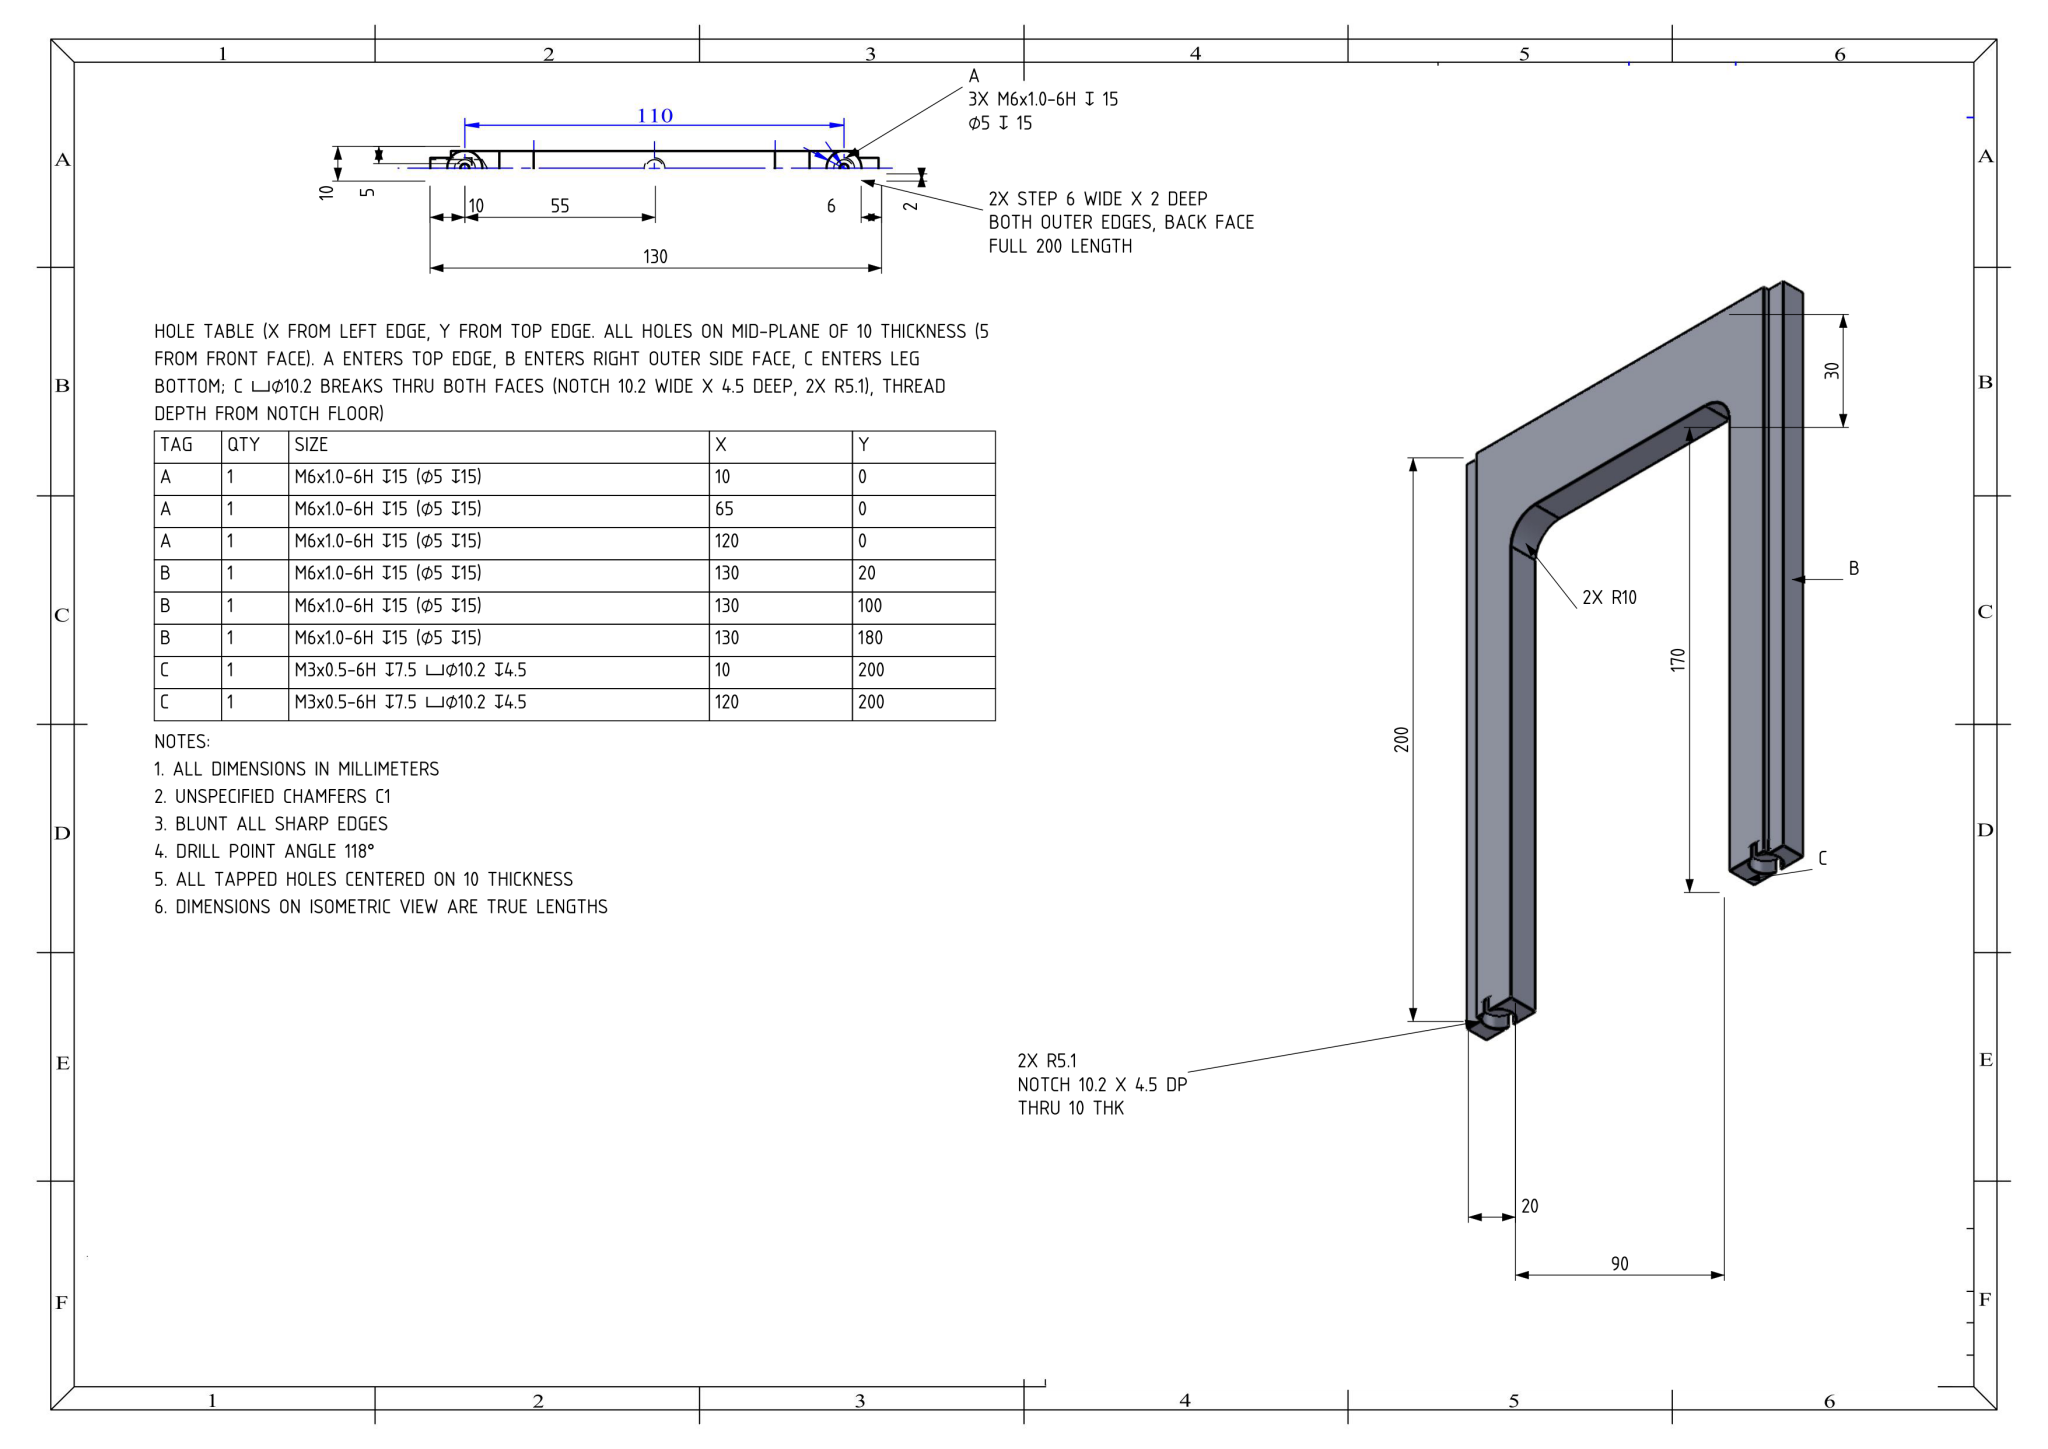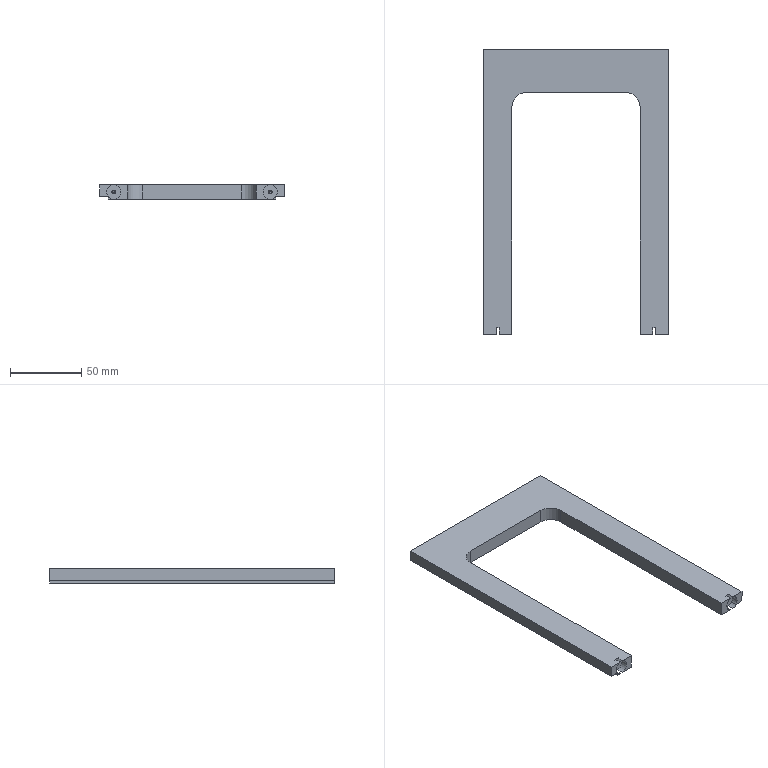Part | NX | mm | 1 solid | 60 faces | box 130 x 200 x 10 mm | volume 99994 mm3 | cylinder 24 | plane 20 | cone 16 | commonest cylinder face diameters 5 x12 10.2 x6 2.5 x4 20 x2